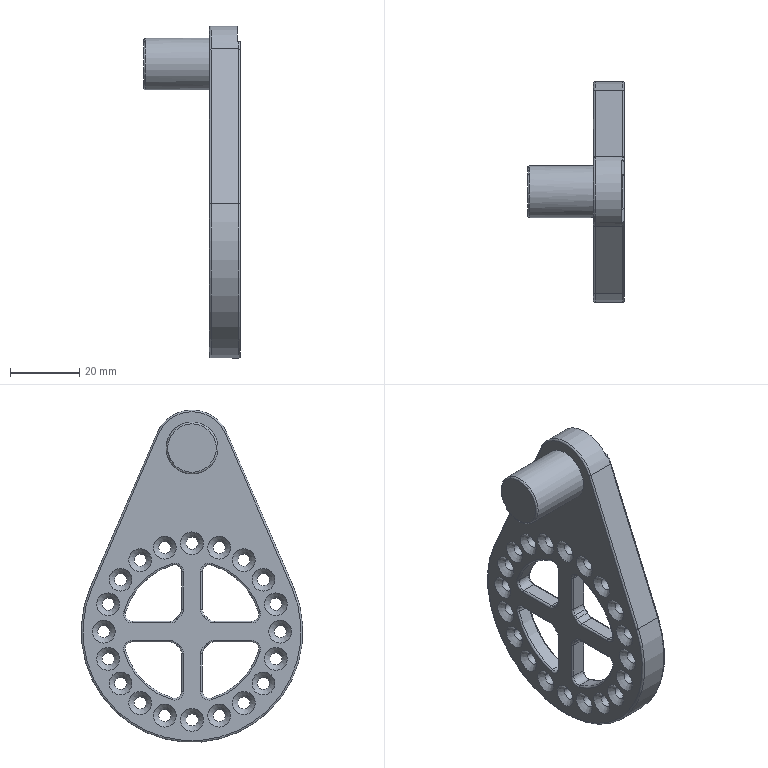Component | NX | MOTOR_DRIVE_ROD | 1 solid | 171 faces | volume 21861 mm3 | cylinder 73 | torus 59 | cone 20 | plane 19 | commonest cylinder face diameters 1 x24 3.5 x20 4 x12 12 x4 4.677 x4 40 x4 64 x1 22 x1